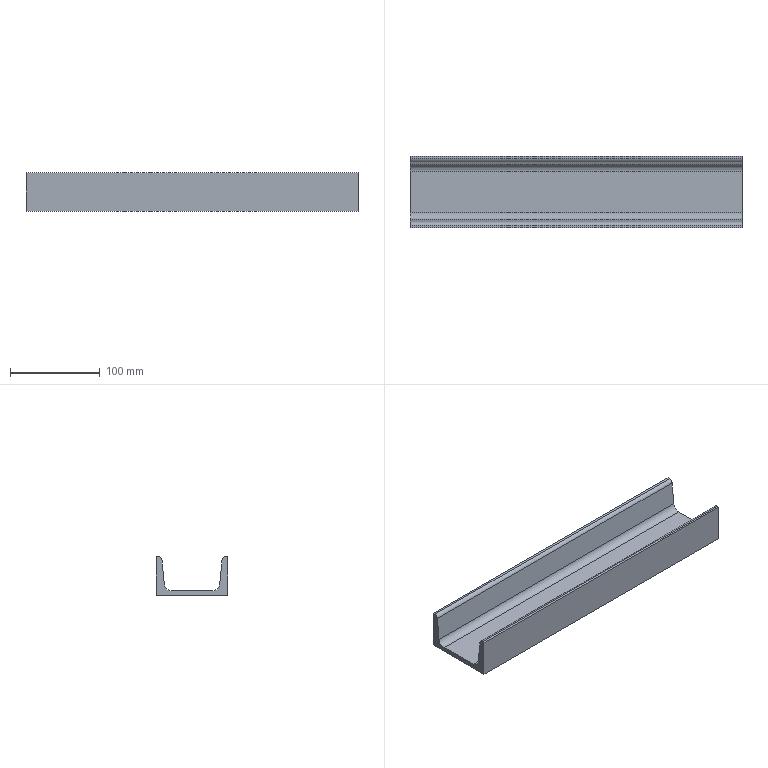Component | SolidWorks | ChannelSteelNo.8470-650-331Machine-1 | 1 solid | 14 faces | box 370 x 80 x 43 mm | volume 378978 mm3 | plane 10 | cylinder 4 | commonest cylinder face diameters 16 x2 8 x2
build123d program:
from build123d import *

# Parameters (mm, degrees)
BOSS_EXTRUDE1_DEPTH = 370


with BuildPart() as part:
    # Sketch1 → Boss-Extrude1 (new body)
    with BuildSketch(Plane(origin=(0, 0, 0), x_dir=(-1, 0, 0), z_dir=(0, 0, -1))):
        with BuildLine():
            Line((-5, 62.86), (-5, 17.14))
            ThreePointArc((-5, 17.14), (-7.068, 11.772), (-12.204, 9.18))
            Line((-12.204, 9.18), (-39.398, 6.46))
            ThreePointArc((-39.398, 6.46), (-41.966, 5.164), (-43, 2.48))
            Line((-43, 2.48), (-43, 0))
            Line((-43, 0), (0, 0))
            Line((0, 0), (0, 80))
            Line((0, 80), (-43, 80))
            Line((-43, 80), (-43, 77.52))
            ThreePointArc((-43, 77.52), (-41.966, 74.836), (-39.398, 73.54))
            Line((-39.398, 73.54), (-12.204, 70.82))
            ThreePointArc((-12.204, 70.82), (-7.068, 68.228), (-5, 62.86))
        make_face()
    extrude(amount=-BOSS_EXTRUDE1_DEPTH)


solid = part.part

# Placed as in the assembly
solid = solid.moved(Location((83.319, 723.438, 720.223), (0, -90, 0)))
STEP:
#1=COLOUR_RGB('',0.7922,0.8196,0.9333);
#2=FILL_AREA_STYLE_COLOUR('',#1);
#3=FILL_AREA_STYLE('',(#2));
#4=SURFACE_STYLE_FILL_AREA(#3);
#5=SURFACE_SIDE_STYLE('',(#4));
#6=SURFACE_STYLE_USAGE(.BOTH.,#5);
#7=PRESENTATION_STYLE_ASSIGNMENT((#6));
#8=CARTESIAN_POINT('',(-11.287,28.843,28.836));
#9=VERTEX_POINT('',#8);
#10=CARTESIAN_POINT('',(-11.287,29.157,28.552));
#11=VERTEX_POINT('',#10);
#12=CARTESIAN_POINT('',(-11.287,29.157,28.867));
#13=DIRECTION('',(1.,0.,0.));
#14=DIRECTION('',(0.,0.,1.));
#15=AXIS2_PLACEMENT_3D('',#12,#13,#14);
#16=CIRCLE('',#15,0.315);
#17=EDGE_CURVE('',#9,#11,#16,.T.);
#18=ORIENTED_EDGE('',*,*,#17,.F.);
#19=CARTESIAN_POINT('',(3.28,28.843,28.836));
#20=VERTEX_POINT('',#19);
#21=CARTESIAN_POINT('',(3.28,28.843,28.836));
#22=DIRECTION('',(-1.,-0.,-0.));
#23=VECTOR('',#22,39.37);
#24=LINE('',#21,#23);
#25=EDGE_CURVE('',#20,#9,#24,.T.);
#26=ORIENTED_EDGE('',*,*,#25,.F.);
#27=CARTESIAN_POINT('',(3.28,29.157,28.552));
#28=VERTEX_POINT('',#27);
#29=CARTESIAN_POINT('',(3.28,29.157,28.867));
#30=DIRECTION('',(1.,0.,0.));
#31=DIRECTION('',(0.,0.,1.));
#32=AXIS2_PLACEMENT_3D('',#29,#30,#31);
#33=CIRCLE('',#32,0.315);
#34=EDGE_CURVE('',#20,#28,#33,.T.);
#35=ORIENTED_EDGE('',*,*,#34,.T.);
#36=CARTESIAN_POINT('',(3.28,29.157,28.552));
#37=DIRECTION('',(-1.,-0.,-0.));
#38=VECTOR('',#37,39.37);
#39=LINE('',#36,#38);
#40=EDGE_CURVE('',#28,#11,#39,.T.);
#41=ORIENTED_EDGE('',*,*,#40,.T.);
#42=EDGE_LOOP('',(#18,#26,#35,#41));
#43=FACE_OUTER_BOUND('',#42,.T.);
#44=CARTESIAN_POINT('',(3.28,29.157,28.867));
#45=DIRECTION('',(-1.,-0.,-0.));
#46=DIRECTION('',(0.,0.,-1.));
#47=AXIS2_PLACEMENT_3D('',#44,#45,#46);
#48=CYLINDRICAL_SURFACE('',#47,0.315);
#49=ADVANCED_FACE('',(#43),#48,.F.);
#50=CARTESIAN_POINT('',(-11.287,28.736,29.906));
#51=VERTEX_POINT('',#50);
#52=CARTESIAN_POINT('',(-11.287,28.736,29.906));
#53=DIRECTION('',(-0.,0.0995,-0.995));
#54=VECTOR('',#53,39.37);
#55=LINE('',#52,#54);
#56=EDGE_CURVE('',#51,#9,#55,.T.);
#57=ORIENTED_EDGE('',*,*,#56,.F.);
#58=CARTESIAN_POINT('',(3.28,28.736,29.906));
#59=VERTEX_POINT('',#58);
#60=CARTESIAN_POINT('',(3.28,28.736,29.906));
#61=DIRECTION('',(-1.,-0.,-0.));
#62=VECTOR('',#61,39.37);
#63=LINE('',#60,#62);
#64=EDGE_CURVE('',#59,#51,#63,.T.);
#65=ORIENTED_EDGE('',*,*,#64,.F.);
#66=CARTESIAN_POINT('',(3.28,28.736,29.906));
#67=DIRECTION('',(-0.,0.0995,-0.995));
#68=VECTOR('',#67,39.37);
#69=LINE('',#66,#68);
#70=EDGE_CURVE('',#59,#20,#69,.T.);
#71=ORIENTED_EDGE('',*,*,#70,.T.);
#72=ORIENTED_EDGE('',*,*,#25,.T.);
#73=EDGE_LOOP('',(#57,#65,#71,#72));
#74=FACE_OUTER_BOUND('',#73,.T.);
#75=CARTESIAN_POINT('',(3.28,28.736,29.906));
#76=DIRECTION('',(-0.,0.995,0.0995));
#77=DIRECTION('',(0.,-0.0995,0.995));
#78=AXIS2_PLACEMENT_3D('',#75,#76,#77);
#79=PLANE('',#78);
#80=ADVANCED_FACE('',(#74),#79,.T.);
#81=CARTESIAN_POINT('',(-11.287,28.579,30.048));
#82=VERTEX_POINT('',#81);
#83=CARTESIAN_POINT('',(-11.287,28.579,29.891));
#84=DIRECTION('',(-1.,-0.,-0.));
#85=DIRECTION('',(0.,0.,-1.));
#86=AXIS2_PLACEMENT_3D('',#83,#84,#85);
#87=CIRCLE('',#86,0.1575);
#88=EDGE_CURVE('',#82,#51,#87,.T.);
#89=ORIENTED_EDGE('',*,*,#88,.F.);
#90=CARTESIAN_POINT('',(3.28,28.579,30.048));
#91=VERTEX_POINT('',#90);
#92=CARTESIAN_POINT('',(3.28,28.579,30.048));
#93=DIRECTION('',(-1.,-0.,-0.));
#94=VECTOR('',#93,39.37);
#95=LINE('',#92,#94);
#96=EDGE_CURVE('',#91,#82,#95,.T.);
#97=ORIENTED_EDGE('',*,*,#96,.F.);
#98=CARTESIAN_POINT('',(3.28,28.579,29.891));
#99=DIRECTION('',(-1.,-0.,-0.));
#100=DIRECTION('',(0.,0.,-1.));
#101=AXIS2_PLACEMENT_3D('',#98,#99,#100);
#102=CIRCLE('',#101,0.1575);
#103=EDGE_CURVE('',#91,#59,#102,.T.);
#104=ORIENTED_EDGE('',*,*,#103,.T.);
#105=ORIENTED_EDGE('',*,*,#64,.T.);
#106=EDGE_LOOP('',(#89,#97,#104,#105));
#107=FACE_OUTER_BOUND('',#106,.T.);
#108=CARTESIAN_POINT('',(3.28,28.579,29.891));
#109=DIRECTION('',(-1.,-0.,-0.));
#110=DIRECTION('',(0.,0.,-1.));
#111=AXIS2_PLACEMENT_3D('',#108,#109,#110);
#112=CYLINDRICAL_SURFACE('',#111,0.1575);
#113=ADVANCED_FACE('',(#107),#112,.T.);
#114=CARTESIAN_POINT('',(-11.287,28.482,30.048));
#115=VERTEX_POINT('',#114);
#116=CARTESIAN_POINT('',(-11.287,28.482,30.048));
#117=DIRECTION('',(-0.,1.,-0.));
#118=VECTOR('',#117,39.37);
#119=LINE('',#116,#118);
#120=EDGE_CURVE('',#115,#82,#119,.T.);
#121=ORIENTED_EDGE('',*,*,#120,.F.);
#122=CARTESIAN_POINT('',(3.28,28.482,30.048));
#123=VERTEX_POINT('',#122);
#124=CARTESIAN_POINT('',(3.28,28.482,30.048));
#125=DIRECTION('',(-1.,-0.,-0.));
#126=VECTOR('',#125,39.37);
#127=LINE('',#124,#126);
#128=EDGE_CURVE('',#123,#115,#127,.T.);
#129=ORIENTED_EDGE('',*,*,#128,.F.);
#130=CARTESIAN_POINT('',(3.28,28.482,30.048));
#131=DIRECTION('',(-0.,1.,-0.));
#132=VECTOR('',#131,39.37);
#133=LINE('',#130,#132);
#134=EDGE_CURVE('',#123,#91,#133,.T.);
#135=ORIENTED_EDGE('',*,*,#134,.T.);
#136=ORIENTED_EDGE('',*,*,#96,.T.);
#137=EDGE_LOOP('',(#121,#129,#135,#136));
#138=FACE_OUTER_BOUND('',#137,.T.);
#139=CARTESIAN_POINT('',(3.28,28.482,30.048));
#140=DIRECTION('',(-0.,-0.,1.));
#141=DIRECTION('',(-1.,-0.,-0.));
#142=AXIS2_PLACEMENT_3D('',#139,#140,#141);
#143=PLANE('',#142);
#144=ADVANCED_FACE('',(#138),#143,.T.);
#145=CARTESIAN_POINT('',(-11.287,28.482,28.355));
#146=VERTEX_POINT('',#145);
#147=CARTESIAN_POINT('',(-11.287,28.482,28.355));
#148=DIRECTION('',(0.,-0.,1.));
#149=VECTOR('',#148,39.37);
#150=LINE('',#147,#149);
#151=EDGE_CURVE('',#146,#115,#150,.T.);
#152=ORIENTED_EDGE('',*,*,#151,.F.);
#153=CARTESIAN_POINT('',(3.28,28.482,28.355));
#154=VERTEX_POINT('',#153);
#155=CARTESIAN_POINT('',(3.28,28.482,28.355));
#156=DIRECTION('',(-1.,-0.,-0.));
#157=VECTOR('',#156,39.37);
#158=LINE('',#155,#157);
#159=EDGE_CURVE('',#154,#146,#158,.T.);
#160=ORIENTED_EDGE('',*,*,#159,.F.);
#161=CARTESIAN_POINT('',(3.28,28.482,28.355));
#162=DIRECTION('',(0.,-0.,1.));
#163=VECTOR('',#162,39.37);
#164=LINE('',#161,#163);
#165=EDGE_CURVE('',#154,#123,#164,.T.);
#166=ORIENTED_EDGE('',*,*,#165,.T.);
#167=ORIENTED_EDGE('',*,*,#128,.T.);
#168=EDGE_LOOP('',(#152,#160,#166,#167));
#169=FACE_OUTER_BOUND('',#168,.T.);
#170=CARTESIAN_POINT('',(3.28,28.482,28.355));
#171=DIRECTION('',(0.,-1.,0.));
#172=DIRECTION('',(1.,0.,0.));
#173=AXIS2_PLACEMENT_3D('',#170,#171,#172);
#174=PLANE('',#173);
#175=ADVANCED_FACE('',(#169),#174,.T.);
#176=CARTESIAN_POINT('',(-11.287,31.631,28.355));
#177=VERTEX_POINT('',#176);
#178=CARTESIAN_POINT('',(-11.287,31.631,28.355));
#179=DIRECTION('',(0.,-1.,0.));
#180=VECTOR('',#179,39.37);
#181=LINE('',#178,#180);
#182=EDGE_CURVE('',#177,#146,#181,.T.);
#183=ORIENTED_EDGE('',*,*,#182,.F.);
#184=CARTESIAN_POINT('',(3.28,31.631,28.355));
#185=VERTEX_POINT('',#184);
#186=CARTESIAN_POINT('',(3.28,31.631,28.355));
#187=DIRECTION('',(-1.,-0.,-0.));
#188=VECTOR('',#187,39.37);
#189=LINE('',#186,#188);
#190=EDGE_CURVE('',#185,#177,#189,.T.);
#191=ORIENTED_EDGE('',*,*,#190,.F.);
#192=CARTESIAN_POINT('',(3.28,31.631,28.355));
#193=DIRECTION('',(0.,-1.,0.));
#194=VECTOR('',#193,39.37);
#195=LINE('',#192,#194);
#196=EDGE_CURVE('',#185,#154,#195,.T.);
#197=ORIENTED_EDGE('',*,*,#196,.T.);
#198=ORIENTED_EDGE('',*,*,#159,.T.);
#199=EDGE_LOOP('',(#183,#191,#197,#198));
#200=FACE_OUTER_BOUND('',#199,.T.);
#201=CARTESIAN_POINT('',(3.28,31.631,28.355));
#202=DIRECTION('',(0.,0.,-1.));
#203=DIRECTION('',(1.,0.,0.));
#204=AXIS2_PLACEMENT_3D('',#201,#202,#203);
#205=PLANE('',#204);
#206=ADVANCED_FACE('',(#200),#205,.T.);
#207=CARTESIAN_POINT('',(-11.287,31.631,30.048));
#208=VERTEX_POINT('',#207);
#209=CARTESIAN_POINT('',(-11.287,31.631,30.048));
#210=DIRECTION('',(-0.,0.,-1.));
#211=VECTOR('',#210,39.37);
#212=LINE('',#209,#211);
#213=EDGE_CURVE('',#208,#177,#212,.T.);
#214=ORIENTED_EDGE('',*,*,#213,.F.);
#215=CARTESIAN_POINT('',(3.28,31.631,30.048));
#216=VERTEX_POINT('',#215);
#217=CARTESIAN_POINT('',(3.28,31.631,30.048));
#218=DIRECTION('',(-1.,-0.,-0.));
#219=VECTOR('',#218,39.37);
#220=LINE('',#217,#219);
#221=EDGE_CURVE('',#216,#208,#220,.T.);
#222=ORIENTED_EDGE('',*,*,#221,.F.);
#223=CARTESIAN_POINT('',(3.28,31.631,30.048));
#224=DIRECTION('',(-0.,0.,-1.));
#225=VECTOR('',#224,39.37);
#226=LINE('',#223,#225);
#227=EDGE_CURVE('',#216,#185,#226,.T.);
#228=ORIENTED_EDGE('',*,*,#227,.T.);
#229=ORIENTED_EDGE('',*,*,#190,.T.);
#230=EDGE_LOOP('',(#214,#222,#228,#229));
#231=FACE_OUTER_BOUND('',#230,.T.);
#232=CARTESIAN_POINT('',(3.28,31.631,30.048));
#233=DIRECTION('',(-0.,1.,-0.));
#234=DIRECTION('',(-1.,-0.,-0.));
#235=AXIS2_PLACEMENT_3D('',#232,#233,#234);
#236=PLANE('',#235);
#237=ADVANCED_FACE('',(#231),#236,.T.);
#238=CARTESIAN_POINT('',(-11.287,31.534,30.048));
#239=VERTEX_POINT('',#238);
#240=CARTESIAN_POINT('',(-11.287,31.534,30.048));
#241=DIRECTION('',(-0.,1.,0.));
#242=VECTOR('',#241,39.37);
#243=LINE('',#240,#242);
#244=EDGE_CURVE('',#239,#208,#243,.T.);
#245=ORIENTED_EDGE('',*,*,#244,.F.);
#246=CARTESIAN_POINT('',(3.28,31.534,30.048));
#247=VERTEX_POINT('',#246);
#248=CARTESIAN_POINT('',(3.28,31.534,30.048));
#249=DIRECTION('',(-1.,-0.,-0.));
#250=VECTOR('',#249,39.37);
#251=LINE('',#248,#250);
#252=EDGE_CURVE('',#247,#239,#251,.T.);
#253=ORIENTED_EDGE('',*,*,#252,.F.);
#254=CARTESIAN_POINT('',(3.28,31.534,30.048));
#255=DIRECTION('',(-0.,1.,0.));
#256=VECTOR('',#255,39.37);
#257=LINE('',#254,#256);
#258=EDGE_CURVE('',#247,#216,#257,.T.);
#259=ORIENTED_EDGE('',*,*,#258,.T.);
#260=ORIENTED_EDGE('',*,*,#221,.T.);
#261=EDGE_LOOP('',(#245,#253,#259,#260));
#262=FACE_OUTER_BOUND('',#261,.T.);
#263=CARTESIAN_POINT('',(3.28,31.534,30.048));
#264=DIRECTION('',(0.,-0.,1.));
#265=DIRECTION('',(0.,-1.,-0.));
#266=AXIS2_PLACEMENT_3D('',#263,#264,#265);
#267=PLANE('',#266);
#268=ADVANCED_FACE('',(#262),#267,.T.);
#269=CARTESIAN_POINT('',(-11.287,31.377,29.906));
#270=VERTEX_POINT('',#269);
#271=CARTESIAN_POINT('',(-11.287,31.534,29.891));
#272=DIRECTION('',(-1.,-0.,-0.));
#273=DIRECTION('',(0.,0.,-1.));
#274=AXIS2_PLACEMENT_3D('',#271,#272,#273);
#275=CIRCLE('',#274,0.1575);
#276=EDGE_CURVE('',#270,#239,#275,.T.);
#277=ORIENTED_EDGE('',*,*,#276,.F.);
#278=CARTESIAN_POINT('',(3.28,31.377,29.906));
#279=VERTEX_POINT('',#278);
#280=CARTESIAN_POINT('',(3.28,31.377,29.906));
#281=DIRECTION('',(-1.,-0.,-0.));
#282=VECTOR('',#281,39.37);
#283=LINE('',#280,#282);
#284=EDGE_CURVE('',#279,#270,#283,.T.);
#285=ORIENTED_EDGE('',*,*,#284,.F.);
#286=CARTESIAN_POINT('',(3.28,31.534,29.891));
#287=DIRECTION('',(-1.,-0.,-0.));
#288=DIRECTION('',(0.,0.,-1.));
#289=AXIS2_PLACEMENT_3D('',#286,#287,#288);
#290=CIRCLE('',#289,0.1575);
#291=EDGE_CURVE('',#279,#247,#290,.T.);
#292=ORIENTED_EDGE('',*,*,#291,.T.);
#293=ORIENTED_EDGE('',*,*,#252,.T.);
#294=EDGE_LOOP('',(#277,#285,#292,#293));
#295=FACE_OUTER_BOUND('',#294,.T.);
#296=CARTESIAN_POINT('',(3.28,31.534,29.891));
#297=DIRECTION('',(-1.,-0.,-0.));
#298=DIRECTION('',(0.,0.,-1.));
#299=AXIS2_PLACEMENT_3D('',#296,#297,#298);
#300=CYLINDRICAL_SURFACE('',#299,0.1575);
#301=ADVANCED_FACE('',(#295),#300,.T.);
#302=CARTESIAN_POINT('',(-11.287,31.27,28.836));
#303=VERTEX_POINT('',#302);
#304=CARTESIAN_POINT('',(-11.287,31.27,28.836));
#305=DIRECTION('',(0.,0.0995,0.995));
#306=VECTOR('',#305,39.37);
#307=LINE('',#304,#306);
#308=EDGE_CURVE('',#303,#270,#307,.T.);
#309=ORIENTED_EDGE('',*,*,#308,.F.);
#310=CARTESIAN_POINT('',(3.28,31.27,28.836));
#311=VERTEX_POINT('',#310);
#312=CARTESIAN_POINT('',(3.28,31.27,28.836));
#313=DIRECTION('',(-1.,-0.,-0.));
#314=VECTOR('',#313,39.37);
#315=LINE('',#312,#314);
#316=EDGE_CURVE('',#311,#303,#315,.T.);
#317=ORIENTED_EDGE('',*,*,#316,.F.);
#318=CARTESIAN_POINT('',(3.28,31.27,28.836));
#319=DIRECTION('',(0.,0.0995,0.995));
#320=VECTOR('',#319,39.37);
#321=LINE('',#318,#320);
#322=EDGE_CURVE('',#311,#279,#321,.T.);
#323=ORIENTED_EDGE('',*,*,#322,.T.);
#324=ORIENTED_EDGE('',*,*,#284,.T.);
#325=EDGE_LOOP('',(#309,#317,#323,#324));
#326=FACE_OUTER_BOUND('',#325,.T.);
#327=CARTESIAN_POINT('',(3.28,31.27,28.836));
#328=DIRECTION('',(0.,-0.995,0.0995));
#329=DIRECTION('',(-0.,-0.0995,-0.995));
#330=AXIS2_PLACEMENT_3D('',#327,#328,#329);
#331=PLANE('',#330);
#332=ADVANCED_FACE('',(#326),#331,.T.);
#333=CARTESIAN_POINT('',(-11.287,30.957,28.552));
#334=VERTEX_POINT('',#333);
#335=CARTESIAN_POINT('',(-11.287,30.957,28.867));
#336=DIRECTION('',(1.,0.,0.));
#337=DIRECTION('',(0.,0.,1.));
#338=AXIS2_PLACEMENT_3D('',#335,#336,#337);
#339=CIRCLE('',#338,0.315);
#340=EDGE_CURVE('',#334,#303,#339,.T.);
#341=ORIENTED_EDGE('',*,*,#340,.F.);
#342=CARTESIAN_POINT('',(3.28,30.957,28.552));
#343=VERTEX_POINT('',#342);
#344=CARTESIAN_POINT('',(3.28,30.957,28.552));
#345=DIRECTION('',(-1.,-0.,-0.));
#346=VECTOR('',#345,39.37);
#347=LINE('',#344,#346);
#348=EDGE_CURVE('',#343,#334,#347,.T.);
#349=ORIENTED_EDGE('',*,*,#348,.F.);
#350=CARTESIAN_POINT('',(3.28,30.957,28.867));
#351=DIRECTION('',(1.,0.,0.));
#352=DIRECTION('',(0.,0.,1.));
#353=AXIS2_PLACEMENT_3D('',#350,#351,#352);
#354=CIRCLE('',#353,0.315);
#355=EDGE_CURVE('',#343,#311,#354,.T.);
#356=ORIENTED_EDGE('',*,*,#355,.T.);
#357=ORIENTED_EDGE('',*,*,#316,.T.);
#358=EDGE_LOOP('',(#341,#349,#356,#357));
#359=FACE_OUTER_BOUND('',#358,.T.);
#360=CARTESIAN_POINT('',(3.28,30.957,28.867));
#361=DIRECTION('',(-1.,-0.,-0.));
#362=DIRECTION('',(0.,0.,-1.));
#363=AXIS2_PLACEMENT_3D('',#360,#361,#362);
#364=CYLINDRICAL_SURFACE('',#363,0.315);
#365=ADVANCED_FACE('',(#359),#364,.F.);
#366=CARTESIAN_POINT('',(-11.287,29.157,28.552));
#367=DIRECTION('',(-0.,1.,-0.));
#368=VECTOR('',#367,39.37);
#369=LINE('',#366,#368);
#370=EDGE_CURVE('',#11,#334,#369,.T.);
#371=ORIENTED_EDGE('',*,*,#370,.F.);
#372=ORIENTED_EDGE('',*,*,#40,.F.);
#373=CARTESIAN_POINT('',(3.28,29.157,28.552));
#374=DIRECTION('',(-0.,1.,-0.));
#375=VECTOR('',#374,39.37);
#376=LINE('',#373,#375);
#377=EDGE_CURVE('',#28,#343,#376,.T.);
#378=ORIENTED_EDGE('',*,*,#377,.T.);
#379=ORIENTED_EDGE('',*,*,#348,.T.);
#380=EDGE_LOOP('',(#371,#372,#378,#379));
#381=FACE_OUTER_BOUND('',#380,.T.);
#382=CARTESIAN_POINT('',(3.28,29.157,28.552));
#383=DIRECTION('',(0.,0.,1.));
#384=DIRECTION('',(0.,-1.,0.));
#385=AXIS2_PLACEMENT_3D('',#382,#383,#384);
#386=PLANE('',#385);
#387=ADVANCED_FACE('',(#381),#386,.T.);
#388=ORIENTED_EDGE('',*,*,#34,.F.);
#389=ORIENTED_EDGE('',*,*,#70,.F.);
#390=ORIENTED_EDGE('',*,*,#103,.F.);
#391=ORIENTED_EDGE('',*,*,#134,.F.);
#392=ORIENTED_EDGE('',*,*,#165,.F.);
#393=ORIENTED_EDGE('',*,*,#196,.F.);
#394=ORIENTED_EDGE('',*,*,#227,.F.);
#395=ORIENTED_EDGE('',*,*,#258,.F.);
#396=ORIENTED_EDGE('',*,*,#291,.F.);
#397=ORIENTED_EDGE('',*,*,#322,.F.);
#398=ORIENTED_EDGE('',*,*,#355,.F.);
#399=ORIENTED_EDGE('',*,*,#377,.F.);
#400=EDGE_LOOP('',(#388,#389,#390,#391,#392,#393,#394,#395,#396,#397,#398,#399));
#401=FACE_OUTER_BOUND('',#400,.T.);
#402=CARTESIAN_POINT('',(3.28,29.157,28.867));
#403=DIRECTION('',(1.,0.,-0.));
#404=DIRECTION('',(0.,-0.,1.));
#405=AXIS2_PLACEMENT_3D('',#402,#403,#404);
#406=PLANE('',#405);
#407=ADVANCED_FACE('',(#401),#406,.T.);
#408=ORIENTED_EDGE('',*,*,#17,.T.);
#409=ORIENTED_EDGE('',*,*,#370,.T.);
#410=ORIENTED_EDGE('',*,*,#340,.T.);
#411=ORIENTED_EDGE('',*,*,#308,.T.);
#412=ORIENTED_EDGE('',*,*,#276,.T.);
#413=ORIENTED_EDGE('',*,*,#244,.T.);
#414=ORIENTED_EDGE('',*,*,#213,.T.);
#415=ORIENTED_EDGE('',*,*,#182,.T.);
#416=ORIENTED_EDGE('',*,*,#151,.T.);
#417=ORIENTED_EDGE('',*,*,#120,.T.);
#418=ORIENTED_EDGE('',*,*,#88,.T.);
#419=ORIENTED_EDGE('',*,*,#56,.T.);
#420=EDGE_LOOP('',(#408,#409,#410,#411,#412,#413,#414,#415,#416,#417,#418,#419));
#421=FACE_OUTER_BOUND('',#420,.T.);
#422=CARTESIAN_POINT('',(-11.287,29.157,28.867));
#423=DIRECTION('',(1.,0.,-0.));
#424=DIRECTION('',(0.,-0.,1.));
#425=AXIS2_PLACEMENT_3D('',#422,#423,#424);
#426=PLANE('',#425);
#427=ADVANCED_FACE('',(#421),#426,.F.);
#428=CLOSED_SHELL('',(#49,#80,#113,#144,#175,#206,#237,#268,#301,#332,#365,#387,#407,#427));
#429=MANIFOLD_SOLID_BREP('',#428);
#430=STYLED_ITEM('',(#7),#429);
#431=(LENGTH_UNIT()NAMED_UNIT(*)SI_UNIT($,.METRE.));
#432=LENGTH_MEASURE_WITH_UNIT(LENGTH_MEASURE(0.0254),#431);
#433=DIMENSIONAL_EXPONENTS(1.,0.,0.,0.,0.,0.,0.);
#434=(CONVERSION_BASED_UNIT('',#432)LENGTH_UNIT()NAMED_UNIT(#433));
#435=UNCERTAINTY_MEASURE_WITH_UNIT(LENGTH_MEASURE(0.00001),#434,'','');
#436=(NAMED_UNIT(*)PLANE_ANGLE_UNIT()SI_UNIT($,.RADIAN.));
#437=(NAMED_UNIT(*)SI_UNIT($,.STERADIAN.)SOLID_ANGLE_UNIT());
#438=(GEOMETRIC_REPRESENTATION_CONTEXT(3)GLOBAL_UNCERTAINTY_ASSIGNED_CONTEXT((#435))GLOBAL_UNIT_ASSIGNED_CONTEXT((#434,#436,#437))REPRESENTATION_CONTEXT('',''));
#439=MECHANICAL_DESIGN_GEOMETRIC_PRESENTATION_REPRESENTATION('',(#430),#438);
#440=CARTESIAN_POINT('',(0.,0.,0.));
#441=DIRECTION('',(0.,0.,1.));
#442=DIRECTION('',(1.,0.,0.));
#443=AXIS2_PLACEMENT_3D('',#440,#441,#442);
#444=(LENGTH_UNIT()NAMED_UNIT(*)SI_UNIT($,.METRE.));
#445=LENGTH_MEASURE_WITH_UNIT(LENGTH_MEASURE(0.0254),#444);
#446=DIMENSIONAL_EXPONENTS(1.,0.,0.,0.,0.,0.,0.);
#447=(CONVERSION_BASED_UNIT('',#445)LENGTH_UNIT()NAMED_UNIT(#446));
#448=UNCERTAINTY_MEASURE_WITH_UNIT(LENGTH_MEASURE(0.00001),#447,'','');
#449=(NAMED_UNIT(*)PLANE_ANGLE_UNIT()SI_UNIT($,.RADIAN.));
#450=(NAMED_UNIT(*)SI_UNIT($,.STERADIAN.)SOLID_ANGLE_UNIT());
#451=(GEOMETRIC_REPRESENTATION_CONTEXT(3)GLOBAL_UNCERTAINTY_ASSIGNED_CONTEXT((#448))GLOBAL_UNIT_ASSIGNED_CONTEXT((#447,#449,#450))REPRESENTATION_CONTEXT('',''));
#452=ADVANCED_BREP_SHAPE_REPRESENTATION('',(#429,#443),#451);
#453=PRESENTATION_LAYER_ASSIGNMENT('','',(#430));